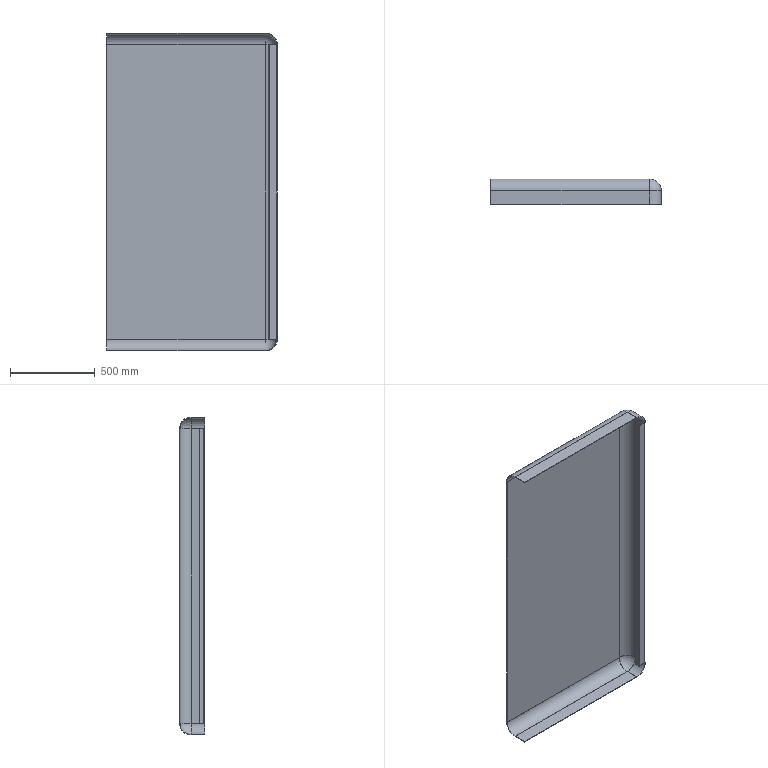Component | SolidWorks | TopHousingAssembly-1_CasingC-1 | 1 solid | 48 faces | volume 7422995 mm3 | plane 30 | cylinder 14 | torus 4 | commonest cylinder face diameters 139 x3 133 x3 4 x2 10 x2 141 x2 135 x2